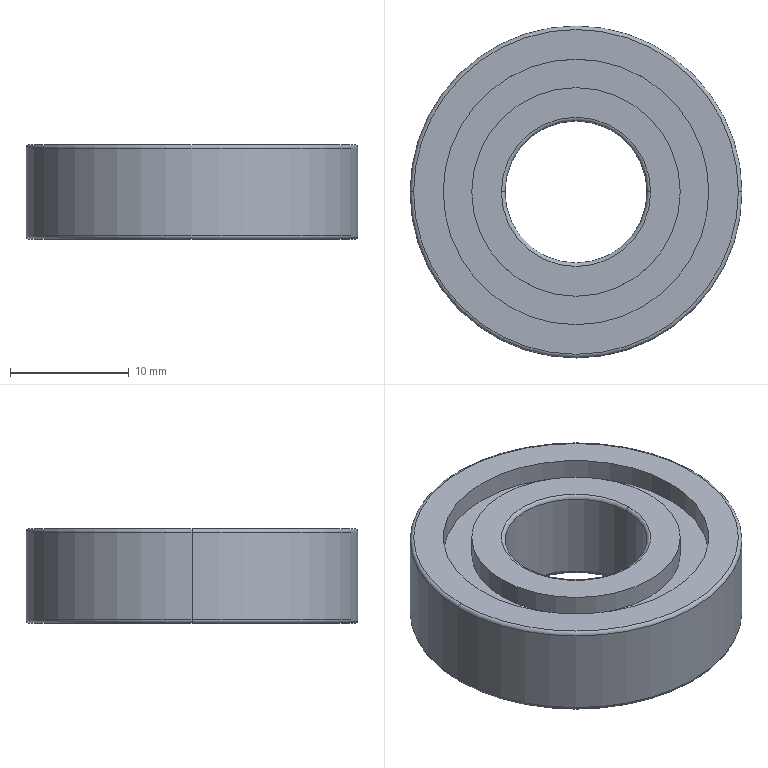Component | SolidWorks | SL010-LeftStreamline-1-1_SL010-2M-0112-000-2-1-1_SL010-B602-1-1 | 1 solid | 32 faces | box 28 x 28 x 8 mm | volume 3620 mm3 | cylinder 16 | torus 8 | plane 8 | commonest cylinder face diameters 22.4 x6 17.6 x6 28 x2 12 x2 | material 45
build123d program:
from build123d import *

# Parameters (mm, degrees)
SKETCH1_W = 0.44
SKETCH1_H = 2.4


with BuildPart() as part:
    # Sketch1 → Revolve1 (revolve)
    with BuildSketch(Plane.XY, mode=Mode.PRIVATE) as revolve1_sk:
        with BuildLine():
            Line((0, 13.7), (0, 11.2))
            Line((0, 11.2), (0.43, 11.2))
            Line((0.43, 11.2), (0.43, 8.8))
            Line((0.43, 8.8), (0, 8.8))
            Line((0, 8.8), (0, 6.3))
            ThreePointArc((0, 6.3), (0.08787, 6.088), (0.3, 6))
            Line((0.3, 6), (7.7, 6))
            ThreePointArc((7.7, 6), (7.912, 6.088), (8, 6.3))
            Line((8, 6.3), (8, 8.8))
            Line((8, 8.8), (6.24, 8.8))
            Line((6.24, 8.8), (6.24, 11.2))
            Line((6.24, 11.2), (8, 11.2))
            Line((8, 11.2), (8, 13.7))
            ThreePointArc((8, 13.7), (7.912, 13.912), (7.7, 14))
            Line((7.7, 14), (0.3, 14))
            ThreePointArc((0.3, 14), (0.08787, 13.912), (0, 13.7))
        make_face()
        with Locations((1.54, 10)):
            Rectangle(SKETCH1_W, SKETCH1_H, mode=Mode.SUBTRACT)
    revolve(revolve1_sk.sketch.rotate(Axis((8, 0, 0), (-1, 0, 0)), 270), axis=Axis((8, 0, 0), (-1, 0, 0)))


solid = part.part

# Placed as in the assembly
solid = solid.moved(Location((-175, -164.904, -666.035), (0, -90, 0)))
STEP:
#1=COLOUR_RGB('',0.7922,0.8196,0.9333);
#2=FILL_AREA_STYLE_COLOUR('',#1);
#3=FILL_AREA_STYLE('',(#2));
#4=SURFACE_STYLE_FILL_AREA(#3);
#5=SURFACE_SIDE_STYLE('',(#4));
#6=SURFACE_STYLE_USAGE(.BOTH.,#5);
#7=PRESENTATION_STYLE_ASSIGNMENT((#6));
#8=CARTESIAN_POINT('',(-7.441,-6.492,-25.919));
#9=VERTEX_POINT('',#8);
#10=CARTESIAN_POINT('',(-6.339,-6.492,-25.919));
#11=VERTEX_POINT('',#10);
#12=CARTESIAN_POINT('',(-6.89,-6.492,-25.919));
#13=DIRECTION('',(0.,0.,-1.));
#14=DIRECTION('',(-1.,0.,0.));
#15=AXIS2_PLACEMENT_3D('',#12,#13,#14);
#16=CIRCLE('',#15,0.5512);
#17=EDGE_CURVE('',#9,#11,#16,.T.);
#18=ORIENTED_EDGE('',*,*,#17,.T.);
#19=CARTESIAN_POINT('',(-6.339,-6.492,-26.21));
#20=VERTEX_POINT('',#19);
#21=CARTESIAN_POINT('',(-6.339,-6.492,-25.907));
#22=DIRECTION('',(0.,0.,-1.));
#23=VECTOR('',#22,39.37);
#24=LINE('',#21,#23);
#25=EDGE_CURVE('',#11,#20,#24,.T.);
#26=ORIENTED_EDGE('',*,*,#25,.T.);
#27=CARTESIAN_POINT('',(-7.441,-6.492,-26.21));
#28=VERTEX_POINT('',#27);
#29=CARTESIAN_POINT('',(-6.89,-6.492,-26.21));
#30=DIRECTION('',(0.,0.,-1.));
#31=DIRECTION('',(-1.,0.,0.));
#32=AXIS2_PLACEMENT_3D('',#29,#30,#31);
#33=CIRCLE('',#32,0.5512);
#34=EDGE_CURVE('',#28,#20,#33,.T.);
#35=ORIENTED_EDGE('',*,*,#34,.F.);
#36=CARTESIAN_POINT('',(-7.441,-6.492,-25.907));
#37=DIRECTION('',(0.,0.,-1.));
#38=VECTOR('',#37,39.37);
#39=LINE('',#36,#38);
#40=EDGE_CURVE('',#9,#28,#39,.T.);
#41=ORIENTED_EDGE('',*,*,#40,.F.);
#42=EDGE_LOOP('',(#18,#26,#35,#41));
#43=FACE_OUTER_BOUND('',#42,.T.);
#44=CARTESIAN_POINT('',(-6.89,-6.492,-25.907));
#45=DIRECTION('',(0.,0.,-1.));
#46=DIRECTION('',(-1.,0.,0.));
#47=AXIS2_PLACEMENT_3D('',#44,#45,#46);
#48=CYLINDRICAL_SURFACE('',#47,0.5512);
#49=ADVANCED_FACE('',(#43),#48,.T.);
#50=CARTESIAN_POINT('',(-7.429,-6.492,-25.907));
#51=VERTEX_POINT('',#50);
#52=CARTESIAN_POINT('',(-6.35,-6.492,-25.907));
#53=VERTEX_POINT('',#52);
#54=CARTESIAN_POINT('',(-6.89,-6.492,-25.907));
#55=DIRECTION('',(0.,0.,-1.));
#56=DIRECTION('',(-1.,0.,0.));
#57=AXIS2_PLACEMENT_3D('',#54,#55,#56);
#58=CIRCLE('',#57,0.5394);
#59=EDGE_CURVE('',#51,#53,#58,.T.);
#60=ORIENTED_EDGE('',*,*,#59,.T.);
#61=CARTESIAN_POINT('',(-6.35,-6.492,-25.919));
#62=DIRECTION('',(0.,1.,0.));
#63=DIRECTION('',(-1.,0.,0.));
#64=AXIS2_PLACEMENT_3D('',#61,#62,#63);
#65=CIRCLE('',#64,0.01181);
#66=EDGE_CURVE('',#53,#11,#65,.T.);
#67=ORIENTED_EDGE('',*,*,#66,.T.);
#68=ORIENTED_EDGE('',*,*,#17,.F.);
#69=CARTESIAN_POINT('',(-7.429,-6.492,-25.919));
#70=DIRECTION('',(-0.,-1.,0.));
#71=DIRECTION('',(1.,0.,0.));
#72=AXIS2_PLACEMENT_3D('',#69,#70,#71);
#73=CIRCLE('',#72,0.01181);
#74=EDGE_CURVE('',#51,#9,#73,.T.);
#75=ORIENTED_EDGE('',*,*,#74,.F.);
#76=EDGE_LOOP('',(#60,#67,#68,#75));
#77=FACE_OUTER_BOUND('',#76,.T.);
#78=CARTESIAN_POINT('',(-6.89,-6.492,-25.919));
#79=DIRECTION('',(0.,0.,-1.));
#80=DIRECTION('',(-1.,0.,0.));
#81=AXIS2_PLACEMENT_3D('',#78,#79,#80);
#82=TOROIDAL_SURFACE('',#81,0.5394,0.01181);
#83=ADVANCED_FACE('',(#77),#82,.T.);
#84=CARTESIAN_POINT('',(-6.449,-6.492,-25.907));
#85=VERTEX_POINT('',#84);
#86=CARTESIAN_POINT('',(-7.331,-6.492,-25.907));
#87=VERTEX_POINT('',#86);
#88=CARTESIAN_POINT('',(-6.89,-6.492,-25.907));
#89=DIRECTION('',(0.,0.,-1.));
#90=DIRECTION('',(-1.,0.,0.));
#91=AXIS2_PLACEMENT_3D('',#88,#89,#90);
#92=CIRCLE('',#91,0.4409);
#93=EDGE_CURVE('',#85,#87,#92,.T.);
#94=ORIENTED_EDGE('',*,*,#93,.F.);
#95=CARTESIAN_POINT('',(-6.449,-6.492,-25.976));
#96=VERTEX_POINT('',#95);
#97=CARTESIAN_POINT('',(-6.449,-6.492,-25.907));
#98=DIRECTION('',(0.,0.,-1.));
#99=VECTOR('',#98,39.37);
#100=LINE('',#97,#99);
#101=EDGE_CURVE('',#85,#96,#100,.T.);
#102=ORIENTED_EDGE('',*,*,#101,.T.);
#103=CARTESIAN_POINT('',(-7.331,-6.492,-25.976));
#104=VERTEX_POINT('',#103);
#105=CARTESIAN_POINT('',(-6.89,-6.492,-25.976));
#106=DIRECTION('',(0.,0.,-1.));
#107=DIRECTION('',(-1.,0.,0.));
#108=AXIS2_PLACEMENT_3D('',#105,#106,#107);
#109=CIRCLE('',#108,0.4409);
#110=EDGE_CURVE('',#96,#104,#109,.T.);
#111=ORIENTED_EDGE('',*,*,#110,.T.);
#112=CARTESIAN_POINT('',(-7.331,-6.492,-25.907));
#113=DIRECTION('',(0.,0.,-1.));
#114=VECTOR('',#113,39.37);
#115=LINE('',#112,#114);
#116=EDGE_CURVE('',#87,#104,#115,.T.);
#117=ORIENTED_EDGE('',*,*,#116,.F.);
#118=EDGE_LOOP('',(#94,#102,#111,#117));
#119=FACE_OUTER_BOUND('',#118,.T.);
#120=CARTESIAN_POINT('',(-6.89,-6.492,-25.907));
#121=DIRECTION('',(0.,0.,-1.));
#122=DIRECTION('',(-1.,0.,0.));
#123=AXIS2_PLACEMENT_3D('',#120,#121,#122);
#124=CYLINDRICAL_SURFACE('',#123,0.4409);
#125=ADVANCED_FACE('',(#119),#124,.F.);
#126=CARTESIAN_POINT('',(-7.236,-6.492,-25.907));
#127=VERTEX_POINT('',#126);
#128=CARTESIAN_POINT('',(-6.543,-6.492,-25.907));
#129=VERTEX_POINT('',#128);
#130=CARTESIAN_POINT('',(-6.89,-6.492,-25.907));
#131=DIRECTION('',(0.,0.,-1.));
#132=DIRECTION('',(-1.,0.,0.));
#133=AXIS2_PLACEMENT_3D('',#130,#131,#132);
#134=CIRCLE('',#133,0.3465);
#135=EDGE_CURVE('',#127,#129,#134,.T.);
#136=ORIENTED_EDGE('',*,*,#135,.T.);
#137=CARTESIAN_POINT('',(-6.543,-6.492,-25.976));
#138=VERTEX_POINT('',#137);
#139=CARTESIAN_POINT('',(-6.543,-6.492,-25.907));
#140=DIRECTION('',(0.,0.,-1.));
#141=VECTOR('',#140,39.37);
#142=LINE('',#139,#141);
#143=EDGE_CURVE('',#129,#138,#142,.T.);
#144=ORIENTED_EDGE('',*,*,#143,.T.);
#145=CARTESIAN_POINT('',(-7.236,-6.492,-25.976));
#146=VERTEX_POINT('',#145);
#147=CARTESIAN_POINT('',(-6.89,-6.492,-25.976));
#148=DIRECTION('',(0.,0.,-1.));
#149=DIRECTION('',(-1.,0.,0.));
#150=AXIS2_PLACEMENT_3D('',#147,#148,#149);
#151=CIRCLE('',#150,0.3465);
#152=EDGE_CURVE('',#146,#138,#151,.T.);
#153=ORIENTED_EDGE('',*,*,#152,.F.);
#154=CARTESIAN_POINT('',(-7.236,-6.492,-25.907));
#155=DIRECTION('',(0.,0.,-1.));
#156=VECTOR('',#155,39.37);
#157=LINE('',#154,#156);
#158=EDGE_CURVE('',#127,#146,#157,.T.);
#159=ORIENTED_EDGE('',*,*,#158,.F.);
#160=EDGE_LOOP('',(#136,#144,#153,#159));
#161=FACE_OUTER_BOUND('',#160,.T.);
#162=CARTESIAN_POINT('',(-6.89,-6.492,-25.907));
#163=DIRECTION('',(0.,0.,-1.));
#164=DIRECTION('',(-1.,0.,0.));
#165=AXIS2_PLACEMENT_3D('',#162,#163,#164);
#166=CYLINDRICAL_SURFACE('',#165,0.3465);
#167=ADVANCED_FACE('',(#161),#166,.T.);
#168=CARTESIAN_POINT('',(-7.126,-6.492,-25.919));
#169=VERTEX_POINT('',#168);
#170=CARTESIAN_POINT('',(-6.654,-6.492,-25.919));
#171=VERTEX_POINT('',#170);
#172=CARTESIAN_POINT('',(-6.89,-6.492,-25.919));
#173=DIRECTION('',(0.,0.,-1.));
#174=DIRECTION('',(-1.,0.,0.));
#175=AXIS2_PLACEMENT_3D('',#172,#173,#174);
#176=CIRCLE('',#175,0.2362);
#177=EDGE_CURVE('',#169,#171,#176,.T.);
#178=ORIENTED_EDGE('',*,*,#177,.T.);
#179=CARTESIAN_POINT('',(-6.642,-6.492,-25.907));
#180=VERTEX_POINT('',#179);
#181=CARTESIAN_POINT('',(-6.642,-6.492,-25.919));
#182=DIRECTION('',(0.,1.,0.));
#183=DIRECTION('',(-1.,0.,0.));
#184=AXIS2_PLACEMENT_3D('',#181,#182,#183);
#185=CIRCLE('',#184,0.01181);
#186=EDGE_CURVE('',#171,#180,#185,.T.);
#187=ORIENTED_EDGE('',*,*,#186,.T.);
#188=CARTESIAN_POINT('',(-7.138,-6.492,-25.907));
#189=VERTEX_POINT('',#188);
#190=CARTESIAN_POINT('',(-6.89,-6.492,-25.907));
#191=DIRECTION('',(0.,0.,-1.));
#192=DIRECTION('',(-1.,0.,0.));
#193=AXIS2_PLACEMENT_3D('',#190,#191,#192);
#194=CIRCLE('',#193,0.248);
#195=EDGE_CURVE('',#189,#180,#194,.T.);
#196=ORIENTED_EDGE('',*,*,#195,.F.);
#197=CARTESIAN_POINT('',(-7.138,-6.492,-25.919));
#198=DIRECTION('',(-0.,-1.,0.));
#199=DIRECTION('',(1.,0.,0.));
#200=AXIS2_PLACEMENT_3D('',#197,#198,#199);
#201=CIRCLE('',#200,0.01181);
#202=EDGE_CURVE('',#169,#189,#201,.T.);
#203=ORIENTED_EDGE('',*,*,#202,.F.);
#204=EDGE_LOOP('',(#178,#187,#196,#203));
#205=FACE_OUTER_BOUND('',#204,.T.);
#206=CARTESIAN_POINT('',(-6.89,-6.492,-25.919));
#207=DIRECTION('',(0.,0.,-1.));
#208=DIRECTION('',(-1.,0.,0.));
#209=AXIS2_PLACEMENT_3D('',#206,#207,#208);
#210=TOROIDAL_SURFACE('',#209,0.248,0.01181);
#211=ADVANCED_FACE('',(#205),#210,.T.);
#212=CARTESIAN_POINT('',(-6.89,-6.492,-25.919));
#213=DIRECTION('',(0.,0.,-1.));
#214=DIRECTION('',(-1.,0.,0.));
#215=AXIS2_PLACEMENT_3D('',#212,#213,#214);
#216=CIRCLE('',#215,0.2362);
#217=EDGE_CURVE('',#171,#169,#216,.T.);
#218=ORIENTED_EDGE('',*,*,#217,.F.);
#219=CARTESIAN_POINT('',(-6.654,-6.492,-26.21));
#220=VERTEX_POINT('',#219);
#221=CARTESIAN_POINT('',(-6.654,-6.492,-25.907));
#222=DIRECTION('',(0.,0.,-1.));
#223=VECTOR('',#222,39.37);
#224=LINE('',#221,#223);
#225=EDGE_CURVE('',#171,#220,#224,.T.);
#226=ORIENTED_EDGE('',*,*,#225,.T.);
#227=CARTESIAN_POINT('',(-7.126,-6.492,-26.21));
#228=VERTEX_POINT('',#227);
#229=CARTESIAN_POINT('',(-6.89,-6.492,-26.21));
#230=DIRECTION('',(0.,0.,-1.));
#231=DIRECTION('',(-1.,0.,0.));
#232=AXIS2_PLACEMENT_3D('',#229,#230,#231);
#233=CIRCLE('',#232,0.2362);
#234=EDGE_CURVE('',#220,#228,#233,.T.);
#235=ORIENTED_EDGE('',*,*,#234,.T.);
#236=CARTESIAN_POINT('',(-7.126,-6.492,-25.907));
#237=DIRECTION('',(0.,0.,-1.));
#238=VECTOR('',#237,39.37);
#239=LINE('',#236,#238);
#240=EDGE_CURVE('',#169,#228,#239,.T.);
#241=ORIENTED_EDGE('',*,*,#240,.F.);
#242=EDGE_LOOP('',(#218,#226,#235,#241));
#243=FACE_OUTER_BOUND('',#242,.T.);
#244=CARTESIAN_POINT('',(-6.89,-6.492,-25.907));
#245=DIRECTION('',(0.,0.,-1.));
#246=DIRECTION('',(-1.,0.,0.));
#247=AXIS2_PLACEMENT_3D('',#244,#245,#246);
#248=CYLINDRICAL_SURFACE('',#247,0.2362);
#249=ADVANCED_FACE('',(#243),#248,.F.);
#250=CARTESIAN_POINT('',(-7.138,-6.492,-26.222));
#251=VERTEX_POINT('',#250);
#252=CARTESIAN_POINT('',(-6.642,-6.492,-26.222));
#253=VERTEX_POINT('',#252);
#254=CARTESIAN_POINT('',(-6.89,-6.492,-26.222));
#255=DIRECTION('',(0.,0.,-1.));
#256=DIRECTION('',(-1.,0.,0.));
#257=AXIS2_PLACEMENT_3D('',#254,#255,#256);
#258=CIRCLE('',#257,0.248);
#259=EDGE_CURVE('',#251,#253,#258,.T.);
#260=ORIENTED_EDGE('',*,*,#259,.T.);
#261=CARTESIAN_POINT('',(-6.642,-6.492,-26.21));
#262=DIRECTION('',(0.,1.,0.));
#263=DIRECTION('',(-1.,0.,0.));
#264=AXIS2_PLACEMENT_3D('',#261,#262,#263);
#265=CIRCLE('',#264,0.01181);
#266=EDGE_CURVE('',#253,#220,#265,.T.);
#267=ORIENTED_EDGE('',*,*,#266,.T.);
#268=CARTESIAN_POINT('',(-6.89,-6.492,-26.21));
#269=DIRECTION('',(0.,0.,-1.));
#270=DIRECTION('',(-1.,0.,0.));
#271=AXIS2_PLACEMENT_3D('',#268,#269,#270);
#272=CIRCLE('',#271,0.2362);
#273=EDGE_CURVE('',#228,#220,#272,.T.);
#274=ORIENTED_EDGE('',*,*,#273,.F.);
#275=CARTESIAN_POINT('',(-7.138,-6.492,-26.21));
#276=DIRECTION('',(-0.,-1.,0.));
#277=DIRECTION('',(1.,0.,0.));
#278=AXIS2_PLACEMENT_3D('',#275,#276,#277);
#279=CIRCLE('',#278,0.01181);
#280=EDGE_CURVE('',#251,#228,#279,.T.);
#281=ORIENTED_EDGE('',*,*,#280,.F.);
#282=EDGE_LOOP('',(#260,#267,#274,#281));
#283=FACE_OUTER_BOUND('',#282,.T.);
#284=CARTESIAN_POINT('',(-6.89,-6.492,-26.21));
#285=DIRECTION('',(0.,0.,-1.));
#286=DIRECTION('',(-1.,0.,0.));
#287=AXIS2_PLACEMENT_3D('',#284,#285,#286);
#288=TOROIDAL_SURFACE('',#287,0.248,0.01181);
#289=ADVANCED_FACE('',(#283),#288,.T.);
#290=CARTESIAN_POINT('',(-7.236,-6.492,-26.205));
#291=VERTEX_POINT('',#290);
#292=CARTESIAN_POINT('',(-6.543,-6.492,-26.205));
#293=VERTEX_POINT('',#292);
#294=CARTESIAN_POINT('',(-6.89,-6.492,-26.205));
#295=DIRECTION('',(0.,0.,-1.));
#296=DIRECTION('',(-1.,0.,0.));
#297=AXIS2_PLACEMENT_3D('',#294,#295,#296);
#298=CIRCLE('',#297,0.3465);
#299=EDGE_CURVE('',#291,#293,#298,.T.);
#300=ORIENTED_EDGE('',*,*,#299,.T.);
#301=CARTESIAN_POINT('',(-6.543,-6.492,-26.222));
#302=VERTEX_POINT('',#301);
#303=CARTESIAN_POINT('',(-6.543,-6.492,-25.907));
#304=DIRECTION('',(0.,0.,-1.));
#305=VECTOR('',#304,39.37);
#306=LINE('',#303,#305);
#307=EDGE_CURVE('',#293,#302,#306,.T.);
#308=ORIENTED_EDGE('',*,*,#307,.T.);
#309=CARTESIAN_POINT('',(-7.236,-6.492,-26.222));
#310=VERTEX_POINT('',#309);
#311=CARTESIAN_POINT('',(-6.89,-6.492,-26.222));
#312=DIRECTION('',(0.,0.,-1.));
#313=DIRECTION('',(-1.,0.,0.));
#314=AXIS2_PLACEMENT_3D('',#311,#312,#313);
#315=CIRCLE('',#314,0.3465);
#316=EDGE_CURVE('',#310,#302,#315,.T.);
#317=ORIENTED_EDGE('',*,*,#316,.F.);
#318=CARTESIAN_POINT('',(-7.236,-6.492,-25.907));
#319=DIRECTION('',(0.,0.,-1.));
#320=VECTOR('',#319,39.37);
#321=LINE('',#318,#320);
#322=EDGE_CURVE('',#291,#310,#321,.T.);
#323=ORIENTED_EDGE('',*,*,#322,.F.);
#324=EDGE_LOOP('',(#300,#308,#317,#323));
#325=FACE_OUTER_BOUND('',#324,.T.);
#326=CARTESIAN_POINT('',(-6.89,-6.492,-25.907));
#327=DIRECTION('',(0.,0.,-1.));
#328=DIRECTION('',(-1.,0.,0.));
#329=AXIS2_PLACEMENT_3D('',#326,#327,#328);
#330=CYLINDRICAL_SURFACE('',#329,0.3465);
#331=ADVANCED_FACE('',(#325),#330,.T.);
#332=CARTESIAN_POINT('',(-6.449,-6.492,-26.205));
#333=VERTEX_POINT('',#332);
#334=CARTESIAN_POINT('',(-7.331,-6.492,-26.205));
#335=VERTEX_POINT('',#334);
#336=CARTESIAN_POINT('',(-6.89,-6.492,-26.205));
#337=DIRECTION('',(0.,0.,-1.));
#338=DIRECTION('',(-1.,0.,0.));
#339=AXIS2_PLACEMENT_3D('',#336,#337,#338);
#340=CIRCLE('',#339,0.4409);
#341=EDGE_CURVE('',#333,#335,#340,.T.);
#342=ORIENTED_EDGE('',*,*,#341,.F.);
#343=CARTESIAN_POINT('',(-6.449,-6.492,-26.222));
#344=VERTEX_POINT('',#343);
#345=CARTESIAN_POINT('',(-6.449,-6.492,-25.907));
#346=DIRECTION('',(0.,0.,-1.));
#347=VECTOR('',#346,39.37);
#348=LINE('',#345,#347);
#349=EDGE_CURVE('',#333,#344,#348,.T.);
#350=ORIENTED_EDGE('',*,*,#349,.T.);
#351=CARTESIAN_POINT('',(-7.331,-6.492,-26.222));
#352=VERTEX_POINT('',#351);
#353=CARTESIAN_POINT('',(-6.89,-6.492,-26.222));
#354=DIRECTION('',(0.,0.,-1.));
#355=DIRECTION('',(-1.,0.,0.));
#356=AXIS2_PLACEMENT_3D('',#353,#354,#355);
#357=CIRCLE('',#356,0.4409);
#358=EDGE_CURVE('',#344,#352,#357,.T.);
#359=ORIENTED_EDGE('',*,*,#358,.T.);
#360=CARTESIAN_POINT('',(-7.331,-6.492,-25.907));
#361=DIRECTION('',(0.,0.,-1.));
#362=VECTOR('',#361,39.37);
#363=LINE('',#360,#362);
#364=EDGE_CURVE('',#335,#352,#363,.T.);
#365=ORIENTED_EDGE('',*,*,#364,.F.);
#366=EDGE_LOOP('',(#342,#350,#359,#365));
#367=FACE_OUTER_BOUND('',#366,.T.);
#368=CARTESIAN_POINT('',(-6.89,-6.492,-25.907));
#369=DIRECTION('',(0.,0.,-1.));
#370=DIRECTION('',(-1.,0.,0.));
#371=AXIS2_PLACEMENT_3D('',#368,#369,#370);
#372=CYLINDRICAL_SURFACE('',#371,0.4409);
#373=ADVANCED_FACE('',(#367),#372,.F.);
#374=ORIENTED_EDGE('',*,*,#34,.T.);
#375=CARTESIAN_POINT('',(-6.35,-6.492,-26.222));
#376=VERTEX_POINT('',#375);
#377=CARTESIAN_POINT('',(-6.35,-6.492,-26.21));
#378=DIRECTION('',(0.,1.,0.));
#379=DIRECTION('',(-1.,0.,0.));
#380=AXIS2_PLACEMENT_3D('',#377,#378,#379);
#381=CIRCLE('',#380,0.01181);
#382=EDGE_CURVE('',#20,#376,#381,.T.);
#383=ORIENTED_EDGE('',*,*,#382,.T.);
#384=CARTESIAN_POINT('',(-7.429,-6.492,-26.222));
#385=VERTEX_POINT('',#384);
#386=CARTESIAN_POINT('',(-6.89,-6.492,-26.222));
#387=DIRECTION('',(0.,0.,-1.));
#388=DIRECTION('',(-1.,0.,0.));
#389=AXIS2_PLACEMENT_3D('',#386,#387,#388);
#390=CIRCLE('',#389,0.5394);
#391=EDGE_CURVE('',#385,#376,#390,.T.);
#392=ORIENTED_EDGE('',*,*,#391,.F.);
#393=CARTESIAN_POINT('',(-7.429,-6.492,-26.21));
#394=DIRECTION('',(-0.,-1.,0.));
#395=DIRECTION('',(1.,0.,0.));
#396=AXIS2_PLACEMENT_3D('',#393,#394,#395);
#397=CIRCLE('',#396,0.01181);
#398=EDGE_CURVE('',#28,#385,#397,.T.);
#399=ORIENTED_EDGE('',*,*,#398,.F.);
#400=EDGE_LOOP('',(#374,#383,#392,#399));
#401=FACE_OUTER_BOUND('',#400,.T.);
#402=CARTESIAN_POINT('',(-6.89,-6.492,-26.21));
#403=DIRECTION('',(0.,0.,-1.));
#404=DIRECTION('',(-1.,0.,0.));
#405=AXIS2_PLACEMENT_3D('',#402,#403,#404);
#406=TOROIDAL_SURFACE('',#405,0.5394,0.01181);
#407=ADVANCED_FACE('',(#401),#406,.T.);
#408=ORIENTED_EDGE('',*,*,#382,.F.);
#409=CARTESIAN_POINT('',(-6.89,-6.492,-26.21));
#410=DIRECTION('',(0.,0.,-1.));
#411=DIRECTION('',(-1.,0.,0.));
#412=AXIS2_PLACEMENT_3D('',#409,#410,#411);
#413=CIRCLE('',#412,0.5512);
#414=EDGE_CURVE('',#20,#28,#413,.T.);
#415=ORIENTED_EDGE('',*,*,#414,.T.);
#416=ORIENTED_EDGE('',*,*,#398,.T.);
#417=CARTESIAN_POINT('',(-6.89,-6.492,-26.222));
#418=DIRECTION('',(0.,0.,-1.));
#419=DIRECTION('',(-1.,0.,0.));
#420=AXIS2_PLACEMENT_3D('',#417,#418,#419);
#421=CIRCLE('',#420,0.5394);
#422=EDGE_CURVE('',#376,#385,#421,.T.);
#423=ORIENTED_EDGE('',*,*,#422,.F.);
#424=EDGE_LOOP('',(#408,#415,#416,#423));
#425=FACE_OUTER_BOUND('',#424,.T.);
#426=CARTESIAN_POINT('',(-6.89,-6.492,-26.21));
#427=DIRECTION('',(0.,0.,-1.));
#428=DIRECTION('',(-1.,0.,0.));
#429=AXIS2_PLACEMENT_3D('',#426,#427,#428);
#430=TOROIDAL_SURFACE('',#429,0.5394,0.01181);
#431=ADVANCED_FACE('',(#425),#430,.T.);
#432=CARTESIAN_POINT('',(-6.89,-6.492,-26.222));
#433=DIRECTION('',(0.,0.,-1.));
#434=DIRECTION('',(-1.,0.,0.));
#435=AXIS2_PLACEMENT_3D('',#432,#433,#434);
#436=CIRCLE('',#435,0.4409);
#437=EDGE_CURVE('',#352,#344,#436,.T.);
#438=ORIENTED_EDGE('',*,*,#437,.F.);
#439=ORIENTED_EDGE('',*,*,#358,.F.);
#440=EDGE_LOOP('',(#438,#439));
#441=FACE_BOUND('',#440,.T.);
#442=ORIENTED_EDGE('',*,*,#391,.T.);
#443=ORIENTED_EDGE('',*,*,#422,.T.);
#444=EDGE_LOOP('',(#442,#443));
#445=FACE_OUTER_BOUND('',#444,.T.);
#446=CARTESIAN_POINT('',(-6.89,-5.953,-26.222));
#447=DIRECTION('',(0.,0.,1.));
#448=DIRECTION('',(1.,-0.,0.));
#449=AXIS2_PLACEMENT_3D('',#446,#447,#448);
#450=PLANE('',#449);
#451=ADVANCED_FACE('',(#441,#445),#450,.F.);
#452=ORIENTED_EDGE('',*,*,#349,.F.);
#453=CARTESIAN_POINT('',(-6.89,-6.492,-26.205));
#454=DIRECTION('',(0.,0.,-1.));
#455=DIRECTION('',(-1.,0.,0.));
#456=AXIS2_PLACEMENT_3D('',#453,#454,#455);
#457=CIRCLE('',#456,0.4409);
#458=EDGE_CURVE('',#335,#333,#457,.T.);
#459=ORIENTED_EDGE('',*,*,#458,.F.);
#460=ORIENTED_EDGE('',*,*,#364,.T.);
#461=ORIENTED_EDGE('',*,*,#437,.T.);
#462=EDGE_LOOP('',(#452,#459,#460,#461));
#463=FACE_OUTER_BOUND('',#462,.T.);
#464=CARTESIAN_POINT('',(-6.89,-6.492,-25.907));
#465=DIRECTION('',(0.,0.,-1.));
#466=DIRECTION('',(-1.,0.,0.));
#467=AXIS2_PLACEMENT_3D('',#464,#465,#466);
#468=CYLINDRICAL_SURFACE('',#467,0.4409);
#469=ADVANCED_FACE('',(#463),#468,.F.);
#470=ORIENTED_EDGE('',*,*,#299,.F.);
#471=CARTESIAN_POINT('',(-6.89,-6.492,-26.205));
#472=DIRECTION('',(0.,0.,-1.));
#473=DIRECTION('',(-1.,0.,0.));
#474=AXIS2_PLACEMENT_3D('',#471,#472,#473);
#475=CIRCLE('',#474,0.3465);
#476=EDGE_CURVE('',#293,#291,#475,.T.);
#477=ORIENTED_EDGE('',*,*,#476,.F.);
#478=EDGE_LOOP('',(#470,#477));
#479=FACE_BOUND('',#478,.T.);
#480=ORIENTED_EDGE('',*,*,#458,.T.);
#481=ORIENTED_EDGE('',*,*,#341,.T.);
#482=EDGE_LOOP('',(#480,#481));
#483=FACE_OUTER_BOUND('',#482,.T.);
#484=CARTESIAN_POINT('',(-6.89,-6.051,-26.205));
#485=DIRECTION('',(0.,0.,1.));
#486=DIRECTION('',(1.,-0.,0.));
#487=AXIS2_PLACEMENT_3D('',#484,#485,#486);
#488=PLANE('',#487);
#489=ADVANCED_FACE('',(#479,#483),#488,.F.);
#490=ORIENTED_EDGE('',*,*,#307,.F.);
#491=ORIENTED_EDGE('',*,*,#476,.T.);
#492=ORIENTED_EDGE('',*,*,#322,.T.);
#493=CARTESIAN_POINT('',(-6.89,-6.492,-26.222));
#494=DIRECTION('',(0.,0.,-1.));
#495=DIRECTION('',(-1.,0.,0.));
#496=AXIS2_PLACEMENT_3D('',#493,#494,#495);
#497=CIRCLE('',#496,0.3465);
#498=EDGE_CURVE('',#302,#310,#497,.T.);
#499=ORIENTED_EDGE('',*,*,#498,.F.);
#500=EDGE_LOOP('',(#490,#491,#492,#499));
#501=FACE_OUTER_BOUND('',#500,.T.);
#502=CARTESIAN_POINT('',(-6.89,-6.492,-25.907));
#503=DIRECTION('',(0.,0.,-1.));
#504=DIRECTION('',(-1.,0.,0.));
#505=AXIS2_PLACEMENT_3D('',#502,#503,#504);
#506=CYLINDRICAL_SURFACE('',#505,0.3465);
#507=ADVANCED_FACE('',(#501),#506,.T.);
#508=ORIENTED_EDGE('',*,*,#259,.F.);
#509=CARTESIAN_POINT('',(-6.89,-6.492,-26.222));
#510=DIRECTION('',(0.,0.,-1.));
#511=DIRECTION('',(-1.,0.,0.));
#512=AXIS2_PLACEMENT_3D('',#509,#510,#511);
#513=CIRCLE('',#512,0.248);
#514=EDGE_CURVE('',#253,#251,#513,.T.);
#515=ORIENTED_EDGE('',*,*,#514,.F.);
#516=EDGE_LOOP('',(#508,#515));
#517=FACE_BOUND('',#516,.T.);
#518=ORIENTED_EDGE('',*,*,#316,.T.);
#519=ORIENTED_EDGE('',*,*,#498,.T.);
#520=EDGE_LOOP('',(#518,#519));
#521=FACE_OUTER_BOUND('',#520,.T.);
#522=CARTESIAN_POINT('',(-6.89,-6.146,-26.222));
#523=DIRECTION('',(0.,0.,1.));
#524=DIRECTION('',(1.,-0.,0.));
#525=AXIS2_PLACEMENT_3D('',#522,#523,#524);
#526=PLANE('',#525);
#527=ADVANCED_FACE('',(#517,#521),#526,.F.);
#528=ORIENTED_EDGE('',*,*,#266,.F.);
#529=ORIENTED_EDGE('',*,*,#514,.T.);
#530=ORIENTED_EDGE('',*,*,#280,.T.);
#531=ORIENTED_EDGE('',*,*,#234,.F.);
#532=EDGE_LOOP('',(#528,#529,#530,#531));
#533=FACE_OUTER_BOUND('',#532,.T.);
#534=CARTESIAN_POINT('',(-6.89,-6.492,-26.21));
#535=DIRECTION('',(0.,0.,-1.));
#536=DIRECTION('',(-1.,0.,0.));
#537=AXIS2_PLACEMENT_3D('',#534,#535,#536);
#538=TOROIDAL_SURFACE('',#537,0.248,0.01181);
#539=ADVANCED_FACE('',(#533),#538,.T.);
#540=ORIENTED_EDGE('',*,*,#225,.F.);
#541=ORIENTED_EDGE('',*,*,#177,.F.);
#542=ORIENTED_EDGE('',*,*,#240,.T.);
#543=ORIENTED_EDGE('',*,*,#273,.T.);
#544=EDGE_LOOP('',(#540,#541,#542,#543));
#545=FACE_OUTER_BOUND('',#544,.T.);
#546=CARTESIAN_POINT('',(-6.89,-6.492,-25.907));
#547=DIRECTION('',(0.,0.,-1.));
#548=DIRECTION('',(-1.,0.,0.));
#549=AXIS2_PLACEMENT_3D('',#546,#547,#548);
#550=CYLINDRICAL_SURFACE('',#549,0.2362);
#551=ADVANCED_FACE('',(#545),#550,.F.);
#552=ORIENTED_EDGE('',*,*,#186,.F.);
#553=ORIENTED_EDGE('',*,*,#217,.T.);
#554=ORIENTED_EDGE('',*,*,#202,.T.);
#555=CARTESIAN_POINT('',(-6.89,-6.492,-25.907));
#556=DIRECTION('',(0.,0.,-1.));
#557=DIRECTION('',(-1.,0.,0.));
#558=AXIS2_PLACEMENT_3D('',#555,#556,#557);
#559=CIRCLE('',#558,0.248);
#560=EDGE_CURVE('',#180,#189,#559,.T.);
#561=ORIENTED_EDGE('',*,*,#560,.F.);
#562=EDGE_LOOP('',(#552,#553,#554,#561));
#563=FACE_OUTER_BOUND('',#562,.T.);
#564=CARTESIAN_POINT('',(-6.89,-6.492,-25.919));
#565=DIRECTION('',(0.,0.,-1.));
#566=DIRECTION('',(-1.,0.,0.));
#567=AXIS2_PLACEMENT_3D('',#564,#565,#566);
#568=TOROIDAL_SURFACE('',#567,0.248,0.01181);
#569=ADVANCED_FACE('',(#563),#568,.T.);
#570=ORIENTED_EDGE('',*,*,#135,.F.);
#571=CARTESIAN_POINT('',(-6.89,-6.492,-25.907));
#572=DIRECTION('',(0.,0.,-1.));
#573=DIRECTION('',(-1.,0.,0.));
#574=AXIS2_PLACEMENT_3D('',#571,#572,#573);
#575=CIRCLE('',#574,0.3465);
#576=EDGE_CURVE('',#129,#127,#575,.T.);
#577=ORIENTED_EDGE('',*,*,#576,.F.);
#578=EDGE_LOOP('',(#570,#577));
#579=FACE_OUTER_BOUND('',#578,.T.);
#580=ORIENTED_EDGE('',*,*,#195,.T.);
#581=ORIENTED_EDGE('',*,*,#560,.T.);
#582=EDGE_LOOP('',(#580,#581));
#583=FACE_BOUND('',#582,.T.);
#584=CARTESIAN_POINT('',(-6.89,-6.244,-25.907));
#585=DIRECTION('',(0.,0.,-1.));
#586=DIRECTION('',(-1.,0.,0.));
#587=AXIS2_PLACEMENT_3D('',#584,#585,#586);
#588=PLANE('',#587);
#589=ADVANCED_FACE('',(#579,#583),#588,.F.);
#590=ORIENTED_EDGE('',*,*,#143,.F.);
#591=ORIENTED_EDGE('',*,*,#576,.T.);
#592=ORIENTED_EDGE('',*,*,#158,.T.);
#593=CARTESIAN_POINT('',(-6.89,-6.492,-25.976));
#594=DIRECTION('',(0.,0.,-1.));
#595=DIRECTION('',(-1.,0.,0.));
#596=AXIS2_PLACEMENT_3D('',#593,#594,#595);
#597=CIRCLE('',#596,0.3465);
#598=EDGE_CURVE('',#138,#146,#597,.T.);
#599=ORIENTED_EDGE('',*,*,#598,.F.);
#600=EDGE_LOOP('',(#590,#591,#592,#599));
#601=FACE_OUTER_BOUND('',#600,.T.);
#602=CARTESIAN_POINT('',(-6.89,-6.492,-25.907));
#603=DIRECTION('',(0.,0.,-1.));
#604=DIRECTION('',(-1.,0.,0.));
#605=AXIS2_PLACEMENT_3D('',#602,#603,#604);
#606=CYLINDRICAL_SURFACE('',#605,0.3465);
#607=ADVANCED_FACE('',(#601),#606,.T.);
#608=CARTESIAN_POINT('',(-6.89,-6.492,-25.976));
#609=DIRECTION('',(0.,0.,-1.));
#610=DIRECTION('',(-1.,0.,0.));
#611=AXIS2_PLACEMENT_3D('',#608,#609,#610);
#612=CIRCLE('',#611,0.4409);
#613=EDGE_CURVE('',#104,#96,#612,.T.);
#614=ORIENTED_EDGE('',*,*,#613,.F.);
#615=ORIENTED_EDGE('',*,*,#110,.F.);
#616=EDGE_LOOP('',(#614,#615));
#617=FACE_OUTER_BOUND('',#616,.T.);
#618=ORIENTED_EDGE('',*,*,#152,.T.);
#619=ORIENTED_EDGE('',*,*,#598,.T.);
#620=EDGE_LOOP('',(#618,#619));
#621=FACE_BOUND('',#620,.T.);
#622=CARTESIAN_POINT('',(-6.89,-6.146,-25.976));
#623=DIRECTION('',(0.,0.,-1.));
#624=DIRECTION('',(-1.,0.,0.));
#625=AXIS2_PLACEMENT_3D('',#622,#623,#624);
#626=PLANE('',#625);
#627=ADVANCED_FACE('',(#617,#621),#626,.F.);
#628=ORIENTED_EDGE('',*,*,#101,.F.);
#629=CARTESIAN_POINT('',(-6.89,-6.492,-25.907));
#630=DIRECTION('',(0.,0.,-1.));
#631=DIRECTION('',(-1.,0.,0.));
#632=AXIS2_PLACEMENT_3D('',#629,#630,#631);
#633=CIRCLE('',#632,0.4409);
#634=EDGE_CURVE('',#87,#85,#633,.T.);
#635=ORIENTED_EDGE('',*,*,#634,.F.);
#636=ORIENTED_EDGE('',*,*,#116,.T.);
#637=ORIENTED_EDGE('',*,*,#613,.T.);
#638=EDGE_LOOP('',(#628,#635,#636,#637));
#639=FACE_OUTER_BOUND('',#638,.T.);
#640=CARTESIAN_POINT('',(-6.89,-6.492,-25.907));
#641=DIRECTION('',(0.,0.,-1.));
#642=DIRECTION('',(-1.,0.,0.));
#643=AXIS2_PLACEMENT_3D('',#640,#641,#642);
#644=CYLINDRICAL_SURFACE('',#643,0.4409);
#645=ADVANCED_FACE('',(#639),#644,.F.);
#646=ORIENTED_EDGE('',*,*,#59,.F.);
#647=CARTESIAN_POINT('',(-6.89,-6.492,-25.907));
#648=DIRECTION('',(0.,0.,-1.));
#649=DIRECTION('',(-1.,0.,0.));
#650=AXIS2_PLACEMENT_3D('',#647,#648,#649);
#651=CIRCLE('',#650,0.5394);
#652=EDGE_CURVE('',#53,#51,#651,.T.);
#653=ORIENTED_EDGE('',*,*,#652,.F.);
#654=EDGE_LOOP('',(#646,#653));
#655=FACE_OUTER_BOUND('',#654,.T.);
#656=ORIENTED_EDGE('',*,*,#634,.T.);
#657=ORIENTED_EDGE('',*,*,#93,.T.);
#658=EDGE_LOOP('',(#656,#657));
#659=FACE_BOUND('',#658,.T.);
#660=CARTESIAN_POINT('',(-6.89,-6.051,-25.907));
#661=DIRECTION('',(0.,0.,-1.));
#662=DIRECTION('',(-1.,0.,0.));
#663=AXIS2_PLACEMENT_3D('',#660,#661,#662);
#664=PLANE('',#663);
#665=ADVANCED_FACE('',(#655,#659),#664,.F.);
#666=ORIENTED_EDGE('',*,*,#66,.F.);
#667=ORIENTED_EDGE('',*,*,#652,.T.);
#668=ORIENTED_EDGE('',*,*,#74,.T.);
#669=CARTESIAN_POINT('',(-6.89,-6.492,-25.919));
#670=DIRECTION('',(0.,0.,-1.));
#671=DIRECTION('',(-1.,0.,0.));
#672=AXIS2_PLACEMENT_3D('',#669,#670,#671);
#673=CIRCLE('',#672,0.5512);
#674=EDGE_CURVE('',#11,#9,#673,.T.);
#675=ORIENTED_EDGE('',*,*,#674,.F.);
#676=EDGE_LOOP('',(#666,#667,#668,#675));
#677=FACE_OUTER_BOUND('',#676,.T.);
#678=CARTESIAN_POINT('',(-6.89,-6.492,-25.919));
#679=DIRECTION('',(0.,0.,-1.));
#680=DIRECTION('',(-1.,0.,0.));
#681=AXIS2_PLACEMENT_3D('',#678,#679,#680);
#682=TOROIDAL_SURFACE('',#681,0.5394,0.01181);
#683=ADVANCED_FACE('',(#677),#682,.T.);
#684=ORIENTED_EDGE('',*,*,#25,.F.);
#685=ORIENTED_EDGE('',*,*,#674,.T.);
#686=ORIENTED_EDGE('',*,*,#40,.T.);
#687=ORIENTED_EDGE('',*,*,#414,.F.);
#688=EDGE_LOOP('',(#684,#685,#686,#687));
#689=FACE_OUTER_BOUND('',#688,.T.);
#690=CARTESIAN_POINT('',(-6.89,-6.492,-25.907));
#691=DIRECTION('',(0.,0.,-1.));
#692=DIRECTION('',(-1.,0.,0.));
#693=AXIS2_PLACEMENT_3D('',#690,#691,#692);
#694=CYLINDRICAL_SURFACE('',#693,0.5512);
#695=ADVANCED_FACE('',(#689),#694,.T.);
#696=CLOSED_SHELL('',(#49,#83,#125,#167,#211,#249,#289,#331,#373,#407,#431,#451,#469,#489,#507,#527,#539,#551,#569,#589,#607,#627,#645,#665,#683,#695));
#697=CARTESIAN_POINT('',(-7.236,-6.492,-26.153));
#698=VERTEX_POINT('',#697);
#699=CARTESIAN_POINT('',(-6.543,-6.492,-26.153));
#700=VERTEX_POINT('',#699);
#701=CARTESIAN_POINT('',(-6.89,-6.492,-26.153));
#702=DIRECTION('',(0.,0.,-1.));
#703=DIRECTION('',(-1.,0.,0.));
#704=AXIS2_PLACEMENT_3D('',#701,#702,#703);
#705=CIRCLE('',#704,0.3465);
#706=EDGE_CURVE('',#698,#700,#705,.T.);
#707=ORIENTED_EDGE('',*,*,#706,.T.);
#708=CARTESIAN_POINT('',(-6.543,-6.492,-26.17));
#709=VERTEX_POINT('',#708);
#710=CARTESIAN_POINT('',(-6.543,-6.492,-25.907));
#711=DIRECTION('',(0.,0.,-1.));
#712=VECTOR('',#711,39.37);
#713=LINE('',#710,#712);
#714=EDGE_CURVE('',#700,#709,#713,.T.);
#715=ORIENTED_EDGE('',*,*,#714,.T.);
#716=CARTESIAN_POINT('',(-7.236,-6.492,-26.17));
#717=VERTEX_POINT('',#716);
#718=CARTESIAN_POINT('',(-6.89,-6.492,-26.17));
#719=DIRECTION('',(0.,0.,-1.));
#720=DIRECTION('',(-1.,0.,0.));
#721=AXIS2_PLACEMENT_3D('',#718,#719,#720);
#722=CIRCLE('',#721,0.3465);
#723=EDGE_CURVE('',#717,#709,#722,.T.);
#724=ORIENTED_EDGE('',*,*,#723,.F.);
#725=CARTESIAN_POINT('',(-7.236,-6.492,-25.907));
#726=DIRECTION('',(0.,0.,-1.));
#727=VECTOR('',#726,39.37);
#728=LINE('',#725,#727);
#729=EDGE_CURVE('',#698,#717,#728,.T.);
#730=ORIENTED_EDGE('',*,*,#729,.F.);
#731=EDGE_LOOP('',(#707,#715,#724,#730));
#732=FACE_OUTER_BOUND('',#731,.T.);
#733=CARTESIAN_POINT('',(-6.89,-6.492,-25.907));
#734=DIRECTION('',(0.,0.,-1.));
#735=DIRECTION('',(-1.,0.,0.));
#736=AXIS2_PLACEMENT_3D('',#733,#734,#735);
#737=CYLINDRICAL_SURFACE('',#736,0.3465);
#738=ADVANCED_FACE('',(#732),#737,.T.);
#739=CARTESIAN_POINT('',(-6.449,-6.492,-26.153));
#740=VERTEX_POINT('',#739);
#741=CARTESIAN_POINT('',(-7.331,-6.492,-26.153));
#742=VERTEX_POINT('',#741);
#743=CARTESIAN_POINT('',(-6.89,-6.492,-26.153));
#744=DIRECTION('',(0.,0.,-1.));
#745=DIRECTION('',(-1.,0.,0.));
#746=AXIS2_PLACEMENT_3D('',#743,#744,#745);
#747=CIRCLE('',#746,0.4409);
#748=EDGE_CURVE('',#740,#742,#747,.T.);
#749=ORIENTED_EDGE('',*,*,#748,.F.);
#750=CARTESIAN_POINT('',(-6.449,-6.492,-26.17));
#751=VERTEX_POINT('',#750);
#752=CARTESIAN_POINT('',(-6.449,-6.492,-25.907));
#753=DIRECTION('',(0.,0.,-1.));
#754=VECTOR('',#753,39.37);
#755=LINE('',#752,#754);
#756=EDGE_CURVE('',#740,#751,#755,.T.);
#757=ORIENTED_EDGE('',*,*,#756,.T.);
#758=CARTESIAN_POINT('',(-7.331,-6.492,-26.17));
#759=VERTEX_POINT('',#758);
#760=CARTESIAN_POINT('',(-6.89,-6.492,-26.17));
#761=DIRECTION('',(0.,0.,-1.));
#762=DIRECTION('',(-1.,0.,0.));
#763=AXIS2_PLACEMENT_3D('',#760,#761,#762);
#764=CIRCLE('',#763,0.4409);
#765=EDGE_CURVE('',#751,#759,#764,.T.);
#766=ORIENTED_EDGE('',*,*,#765,.T.);
#767=CARTESIAN_POINT('',(-7.331,-6.492,-25.907));
#768=DIRECTION('',(0.,0.,-1.));
#769=VECTOR('',#768,39.37);
#770=LINE('',#767,#769);
#771=EDGE_CURVE('',#742,#759,#770,.T.);
#772=ORIENTED_EDGE('',*,*,#771,.F.);
#773=EDGE_LOOP('',(#749,#757,#766,#772));
#774=FACE_OUTER_BOUND('',#773,.T.);
#775=CARTESIAN_POINT('',(-6.89,-6.492,-25.907));
#776=DIRECTION('',(0.,0.,-1.));
#777=DIRECTION('',(-1.,0.,0.));
#778=AXIS2_PLACEMENT_3D('',#775,#776,#777);
#779=CYLINDRICAL_SURFACE('',#778,0.4409);
#780=ADVANCED_FACE('',(#774),#779,.F.);
#781=ORIENTED_EDGE('',*,*,#756,.F.);
#782=CARTESIAN_POINT('',(-6.89,-6.492,-26.153));
#783=DIRECTION('',(0.,0.,-1.));
#784=DIRECTION('',(-1.,0.,0.));
#785=AXIS2_PLACEMENT_3D('',#782,#783,#784);
#786=CIRCLE('',#785,0.4409);
#787=EDGE_CURVE('',#742,#740,#786,.T.);
#788=ORIENTED_EDGE('',*,*,#787,.F.);
#789=ORIENTED_EDGE('',*,*,#771,.T.);
#790=CARTESIAN_POINT('',(-6.89,-6.492,-26.17));
#791=DIRECTION('',(0.,0.,-1.));
#792=DIRECTION('',(-1.,0.,0.));
#793=AXIS2_PLACEMENT_3D('',#790,#791,#792);
#794=CIRCLE('',#793,0.4409);
#795=EDGE_CURVE('',#759,#751,#794,.T.);
#796=ORIENTED_EDGE('',*,*,#795,.T.);
#797=EDGE_LOOP('',(#781,#788,#789,#796));
#798=FACE_OUTER_BOUND('',#797,.T.);
#799=CARTESIAN_POINT('',(-6.89,-6.492,-25.907));
#800=DIRECTION('',(0.,0.,-1.));
#801=DIRECTION('',(-1.,0.,0.));
#802=AXIS2_PLACEMENT_3D('',#799,#800,#801);
#803=CYLINDRICAL_SURFACE('',#802,0.4409);
#804=ADVANCED_FACE('',(#798),#803,.F.);
#805=ORIENTED_EDGE('',*,*,#787,.T.);
#806=ORIENTED_EDGE('',*,*,#748,.T.);
#807=EDGE_LOOP('',(#805,#806));
#808=FACE_OUTER_BOUND('',#807,.T.);
#809=ORIENTED_EDGE('',*,*,#706,.F.);
#810=CARTESIAN_POINT('',(-6.89,-6.492,-26.153));
#811=DIRECTION('',(0.,0.,-1.));
#812=DIRECTION('',(-1.,0.,0.));
#813=AXIS2_PLACEMENT_3D('',#810,#811,#812);
#814=CIRCLE('',#813,0.3465);
#815=EDGE_CURVE('',#700,#698,#814,.T.);
#816=ORIENTED_EDGE('',*,*,#815,.F.);
#817=EDGE_LOOP('',(#809,#816));
#818=FACE_BOUND('',#817,.T.);
#819=CARTESIAN_POINT('',(-6.89,-6.146,-26.153));
#820=DIRECTION('',(0.,0.,-1.));
#821=DIRECTION('',(-1.,0.,0.));
#822=AXIS2_PLACEMENT_3D('',#819,#820,#821);
#823=PLANE('',#822);
#824=ADVANCED_FACE('',(#808,#818),#823,.T.);
#825=ORIENTED_EDGE('',*,*,#714,.F.);
#826=ORIENTED_EDGE('',*,*,#815,.T.);
#827=ORIENTED_EDGE('',*,*,#729,.T.);
#828=CARTESIAN_POINT('',(-6.89,-6.492,-26.17));
#829=DIRECTION('',(0.,0.,-1.));
#830=DIRECTION('',(-1.,0.,0.));
#831=AXIS2_PLACEMENT_3D('',#828,#829,#830);
#832=CIRCLE('',#831,0.3465);
#833=EDGE_CURVE('',#709,#717,#832,.T.);
#834=ORIENTED_EDGE('',*,*,#833,.F.);
#835=EDGE_LOOP('',(#825,#826,#827,#834));
#836=FACE_OUTER_BOUND('',#835,.T.);
#837=CARTESIAN_POINT('',(-6.89,-6.492,-25.907));
#838=DIRECTION('',(0.,0.,-1.));
#839=DIRECTION('',(-1.,0.,0.));
#840=AXIS2_PLACEMENT_3D('',#837,#838,#839);
#841=CYLINDRICAL_SURFACE('',#840,0.3465);
#842=ADVANCED_FACE('',(#836),#841,.T.);
#843=ORIENTED_EDGE('',*,*,#723,.T.);
#844=ORIENTED_EDGE('',*,*,#833,.T.);
#845=EDGE_LOOP('',(#843,#844));
#846=FACE_BOUND('',#845,.T.);
#847=ORIENTED_EDGE('',*,*,#795,.F.);
#848=ORIENTED_EDGE('',*,*,#765,.F.);
#849=EDGE_LOOP('',(#847,#848));
#850=FACE_OUTER_BOUND('',#849,.T.);
#851=CARTESIAN_POINT('',(-6.89,-6.051,-26.17));
#852=DIRECTION('',(0.,0.,1.));
#853=DIRECTION('',(1.,-0.,0.));
#854=AXIS2_PLACEMENT_3D('',#851,#852,#853);
#855=PLANE('',#854);
#856=ADVANCED_FACE('',(#846,#850),#855,.T.);
#857=CLOSED_SHELL('',(#738,#780,#804,#824,#842,#856));
#858=ORIENTED_CLOSED_SHELL('',*,#857,.F.);
#859=BREP_WITH_VOIDS('',#696,(#858));
#860=STYLED_ITEM('',(#7),#859);
#861=(LENGTH_UNIT()NAMED_UNIT(*)SI_UNIT($,.METRE.));
#862=LENGTH_MEASURE_WITH_UNIT(LENGTH_MEASURE(0.0254),#861);
#863=DIMENSIONAL_EXPONENTS(1.,0.,0.,0.,0.,0.,0.);
#864=(CONVERSION_BASED_UNIT('',#862)LENGTH_UNIT()NAMED_UNIT(#863));
#865=UNCERTAINTY_MEASURE_WITH_UNIT(LENGTH_MEASURE(0.00001),#864,'','');
#866=(NAMED_UNIT(*)PLANE_ANGLE_UNIT()SI_UNIT($,.RADIAN.));
#867=(NAMED_UNIT(*)SI_UNIT($,.STERADIAN.)SOLID_ANGLE_UNIT());
#868=(GEOMETRIC_REPRESENTATION_CONTEXT(3)GLOBAL_UNCERTAINTY_ASSIGNED_CONTEXT((#865))GLOBAL_UNIT_ASSIGNED_CONTEXT((#864,#866,#867))REPRESENTATION_CONTEXT('',''));
#869=MECHANICAL_DESIGN_GEOMETRIC_PRESENTATION_REPRESENTATION('',(#860),#868);
#870=CARTESIAN_POINT('',(0.,0.,0.));
#871=DIRECTION('',(0.,0.,1.));
#872=DIRECTION('',(1.,0.,0.));
#873=AXIS2_PLACEMENT_3D('',#870,#871,#872);
#874=(LENGTH_UNIT()NAMED_UNIT(*)SI_UNIT($,.METRE.));
#875=LENGTH_MEASURE_WITH_UNIT(LENGTH_MEASURE(0.0254),#874);
#876=DIMENSIONAL_EXPONENTS(1.,0.,0.,0.,0.,0.,0.);
#877=(CONVERSION_BASED_UNIT('',#875)LENGTH_UNIT()NAMED_UNIT(#876));
#878=UNCERTAINTY_MEASURE_WITH_UNIT(LENGTH_MEASURE(0.00001),#877,'','');
#879=(NAMED_UNIT(*)PLANE_ANGLE_UNIT()SI_UNIT($,.RADIAN.));
#880=(NAMED_UNIT(*)SI_UNIT($,.STERADIAN.)SOLID_ANGLE_UNIT());
#881=(GEOMETRIC_REPRESENTATION_CONTEXT(3)GLOBAL_UNCERTAINTY_ASSIGNED_CONTEXT((#878))GLOBAL_UNIT_ASSIGNED_CONTEXT((#877,#879,#880))REPRESENTATION_CONTEXT('',''));
#882=ADVANCED_BREP_SHAPE_REPRESENTATION('',(#859,#873),#881);
#883=PRESENTATION_LAYER_ASSIGNMENT('','',(#860));